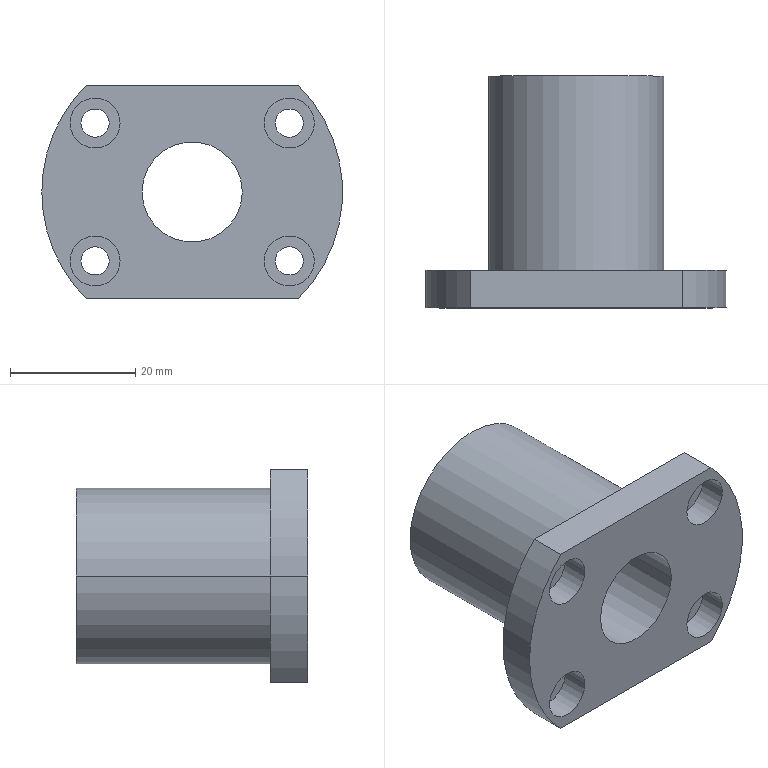Component | SolidWorks | FlangeLinearBearingLMH16UU-1 | 1 solid | 32 faces | box 48 x 37 x 34 mm | volume 19559 mm3 | cylinder 23 | plane 9 | commonest cylinder face diameters 8 x8 4.5 x8 48 x3 16 x2 28 x2
build123d program:
from build123d import *

# Parameters (mm, degrees)
BOSS_EXTRUDE1_DEPTH = 6
SKETCH3_R           = 14
BOSS_EXTRUDE2_DEPTH = 31
SKETCH4_R           = 8
CUT_EXTRUDE1_DEPTH  = 48.265
SKETCH5_R           = 2.25
CUT_EXTRUDE2_DEPTH  = 31
SKETCH6_R           = 4
CUT_EXTRUDE3_DEPTH  = 4.4


with BuildPart() as part:
    # Sketch1 → Boss-Extrude1 (new body)
    with BuildSketch(Plane(origin=(0, 0, 0), x_dir=(1, 0, 0), z_dir=(0, 1, 0))):
        with BuildLine():
            Line((-17, 16.941), (-17, -16.941))
            ThreePointArc((-17, -16.941), (0, -24), (17, -16.941))
            Line((17, -16.941), (17, 16.941))
            ThreePointArc((17, 16.941), (0, 24), (-17, 16.941))
        make_face()
    extrude(amount=BOSS_EXTRUDE1_DEPTH)

    # Sketch3 → Boss-Extrude2 (add)
    with BuildSketch(Plane(origin=(0, 6, 0), x_dir=(1, 0, 0), z_dir=(0, 1, 0))):
        with Locations(Location((0, 0, 0), (0, 0, 270))):
            Circle(SKETCH3_R)
    extrude(amount=BOSS_EXTRUDE2_DEPTH)

    # Sketch4 → Cut-Extrude1 (cut, through all)
    with BuildSketch(Plane(origin=(0, 37, 0), x_dir=(1, 0, 0), z_dir=(0, 1, 0))):
        with Locations(Location((0, 0, 0), (0, 0, 270))):
            Circle(SKETCH4_R)
    extrude(amount=-CUT_EXTRUDE1_DEPTH, mode=Mode.SUBTRACT)

    # Sketch5 → Cut-Extrude2 (cut)
    with BuildSketch(Plane.XZ):
        with Locations(Location((-11, 15.5, 0), (0, 0, 270))):
            Circle(SKETCH5_R)
        with Locations(Location((11, 15.5, 0), (0, 0, 270))):
            Circle(SKETCH5_R)
        with Locations(Location((11, -15.5, 0), (0, 0, 270))):
            Circle(SKETCH5_R)
        with Locations(Location((-11, -15.5, 0), (0, 0, 270))):
            Circle(SKETCH5_R)
    extrude(amount=-CUT_EXTRUDE2_DEPTH, mode=Mode.SUBTRACT)

    # Sketch6 → Cut-Extrude3 (cut)
    with BuildSketch(Plane.XZ):
        with Locations(Location((-11, 15.5, 0), (0, 0, 270))):
            Circle(SKETCH6_R)
        with Locations(Location((11, 15.5, 0), (0, 0, 270))):
            Circle(SKETCH6_R)
        with Locations(Location((11, -15.5, 0), (0, 0, 270))):
            Circle(SKETCH6_R)
        with Locations(Location((-11, -15.5, 0), (0, 0, 270))):
            Circle(SKETCH6_R)
    extrude(amount=-CUT_EXTRUDE3_DEPTH, mode=Mode.SUBTRACT)


solid = part.part

# Placed as in the assembly
solid = solid.moved(Location((32.2, 65.857, 29.75), (0, 90, 0)))
STEP:
#1=CARTESIAN_POINT('',(0.8149,2.766,1.604));
#2=VERTEX_POINT('',#1);
#3=CARTESIAN_POINT('',(0.5,2.766,1.604));
#4=VERTEX_POINT('',#3);
#5=CARTESIAN_POINT('',(0.6575,2.766,1.604));
#6=DIRECTION('',(0.,-1.,0.));
#7=DIRECTION('',(-1.,0.,0.));
#8=AXIS2_PLACEMENT_3D('',#5,#6,#7);
#9=CIRCLE('',#8,0.1575);
#10=EDGE_CURVE('',#2,#4,#9,.T.);
#11=ORIENTED_EDGE('',*,*,#10,.F.);
#12=CARTESIAN_POINT('',(0.8149,2.593,1.604));
#13=VERTEX_POINT('',#12);
#14=CARTESIAN_POINT('',(0.8149,2.766,1.604));
#15=DIRECTION('',(0.,-1.,0.));
#16=VECTOR('',#15,39.37);
#17=LINE('',#14,#16);
#18=EDGE_CURVE('',#2,#13,#17,.T.);
#19=ORIENTED_EDGE('',*,*,#18,.T.);
#20=CARTESIAN_POINT('',(0.5,2.593,1.604));
#21=VERTEX_POINT('',#20);
#22=CARTESIAN_POINT('',(0.6575,2.593,1.604));
#23=DIRECTION('',(0.,-1.,0.));
#24=DIRECTION('',(-1.,0.,0.));
#25=AXIS2_PLACEMENT_3D('',#22,#23,#24);
#26=CIRCLE('',#25,0.1575);
#27=EDGE_CURVE('',#13,#21,#26,.T.);
#28=ORIENTED_EDGE('',*,*,#27,.T.);
#29=CARTESIAN_POINT('',(0.5,2.766,1.604));
#30=DIRECTION('',(0.,-1.,0.));
#31=VECTOR('',#30,39.37);
#32=LINE('',#29,#31);
#33=EDGE_CURVE('',#4,#21,#32,.T.);
#34=ORIENTED_EDGE('',*,*,#33,.F.);
#35=EDGE_LOOP('',(#11,#19,#28,#34));
#36=FACE_OUTER_BOUND('',#35,.T.);
#37=CARTESIAN_POINT('',(0.6575,2.766,1.604));
#38=DIRECTION('',(0.,-1.,0.));
#39=DIRECTION('',(-1.,0.,0.));
#40=AXIS2_PLACEMENT_3D('',#37,#38,#39);
#41=CYLINDRICAL_SURFACE('',#40,0.1575);
#42=ADVANCED_FACE('',(#36),#41,.F.);
#43=CARTESIAN_POINT('',(0.8149,2.766,0.7382));
#44=VERTEX_POINT('',#43);
#45=CARTESIAN_POINT('',(0.5,2.766,0.7382));
#46=VERTEX_POINT('',#45);
#47=CARTESIAN_POINT('',(0.6575,2.766,0.7382));
#48=DIRECTION('',(0.,-1.,0.));
#49=DIRECTION('',(-1.,0.,0.));
#50=AXIS2_PLACEMENT_3D('',#47,#48,#49);
#51=CIRCLE('',#50,0.1575);
#52=EDGE_CURVE('',#44,#46,#51,.T.);
#53=ORIENTED_EDGE('',*,*,#52,.F.);
#54=CARTESIAN_POINT('',(0.8149,2.593,0.7382));
#55=VERTEX_POINT('',#54);
#56=CARTESIAN_POINT('',(0.8149,2.766,0.7382));
#57=DIRECTION('',(0.,-1.,0.));
#58=VECTOR('',#57,39.37);
#59=LINE('',#56,#58);
#60=EDGE_CURVE('',#44,#55,#59,.T.);
#61=ORIENTED_EDGE('',*,*,#60,.T.);
#62=CARTESIAN_POINT('',(0.5,2.593,0.7382));
#63=VERTEX_POINT('',#62);
#64=CARTESIAN_POINT('',(0.6575,2.593,0.7382));
#65=DIRECTION('',(0.,-1.,0.));
#66=DIRECTION('',(-1.,0.,0.));
#67=AXIS2_PLACEMENT_3D('',#64,#65,#66);
#68=CIRCLE('',#67,0.1575);
#69=EDGE_CURVE('',#55,#63,#68,.T.);
#70=ORIENTED_EDGE('',*,*,#69,.T.);
#71=CARTESIAN_POINT('',(0.5,2.766,0.7382));
#72=DIRECTION('',(0.,-1.,0.));
#73=VECTOR('',#72,39.37);
#74=LINE('',#71,#73);
#75=EDGE_CURVE('',#46,#63,#74,.T.);
#76=ORIENTED_EDGE('',*,*,#75,.F.);
#77=EDGE_LOOP('',(#53,#61,#70,#76));
#78=FACE_OUTER_BOUND('',#77,.T.);
#79=CARTESIAN_POINT('',(0.6575,2.766,0.7382));
#80=DIRECTION('',(0.,-1.,0.));
#81=DIRECTION('',(-1.,0.,0.));
#82=AXIS2_PLACEMENT_3D('',#79,#80,#81);
#83=CYLINDRICAL_SURFACE('',#82,0.1575);
#84=ADVANCED_FACE('',(#78),#83,.F.);
#85=CARTESIAN_POINT('',(2.035,2.766,0.7382));
#86=VERTEX_POINT('',#85);
#87=CARTESIAN_POINT('',(1.72,2.766,0.7382));
#88=VERTEX_POINT('',#87);
#89=CARTESIAN_POINT('',(1.878,2.766,0.7382));
#90=DIRECTION('',(0.,-1.,0.));
#91=DIRECTION('',(-1.,0.,0.));
#92=AXIS2_PLACEMENT_3D('',#89,#90,#91);
#93=CIRCLE('',#92,0.1575);
#94=EDGE_CURVE('',#86,#88,#93,.T.);
#95=ORIENTED_EDGE('',*,*,#94,.F.);
#96=CARTESIAN_POINT('',(2.035,2.593,0.7382));
#97=VERTEX_POINT('',#96);
#98=CARTESIAN_POINT('',(2.035,2.766,0.7382));
#99=DIRECTION('',(0.,-1.,0.));
#100=VECTOR('',#99,39.37);
#101=LINE('',#98,#100);
#102=EDGE_CURVE('',#86,#97,#101,.T.);
#103=ORIENTED_EDGE('',*,*,#102,.T.);
#104=CARTESIAN_POINT('',(1.72,2.593,0.7382));
#105=VERTEX_POINT('',#104);
#106=CARTESIAN_POINT('',(1.878,2.593,0.7382));
#107=DIRECTION('',(0.,-1.,0.));
#108=DIRECTION('',(-1.,0.,0.));
#109=AXIS2_PLACEMENT_3D('',#106,#107,#108);
#110=CIRCLE('',#109,0.1575);
#111=EDGE_CURVE('',#97,#105,#110,.T.);
#112=ORIENTED_EDGE('',*,*,#111,.T.);
#113=CARTESIAN_POINT('',(1.72,2.766,0.7382));
#114=DIRECTION('',(0.,-1.,0.));
#115=VECTOR('',#114,39.37);
#116=LINE('',#113,#115);
#117=EDGE_CURVE('',#88,#105,#116,.T.);
#118=ORIENTED_EDGE('',*,*,#117,.F.);
#119=EDGE_LOOP('',(#95,#103,#112,#118));
#120=FACE_OUTER_BOUND('',#119,.T.);
#121=CARTESIAN_POINT('',(1.878,2.766,0.7382));
#122=DIRECTION('',(0.,-1.,0.));
#123=DIRECTION('',(-1.,0.,0.));
#124=AXIS2_PLACEMENT_3D('',#121,#122,#123);
#125=CYLINDRICAL_SURFACE('',#124,0.1575);
#126=ADVANCED_FACE('',(#120),#125,.F.);
#127=CARTESIAN_POINT('',(2.035,2.766,1.604));
#128=VERTEX_POINT('',#127);
#129=CARTESIAN_POINT('',(1.72,2.766,1.604));
#130=VERTEX_POINT('',#129);
#131=CARTESIAN_POINT('',(1.878,2.766,1.604));
#132=DIRECTION('',(0.,-1.,0.));
#133=DIRECTION('',(-1.,0.,0.));
#134=AXIS2_PLACEMENT_3D('',#131,#132,#133);
#135=CIRCLE('',#134,0.1575);
#136=EDGE_CURVE('',#128,#130,#135,.T.);
#137=ORIENTED_EDGE('',*,*,#136,.F.);
#138=CARTESIAN_POINT('',(2.035,2.593,1.604));
#139=VERTEX_POINT('',#138);
#140=CARTESIAN_POINT('',(2.035,2.766,1.604));
#141=DIRECTION('',(0.,-1.,0.));
#142=VECTOR('',#141,39.37);
#143=LINE('',#140,#142);
#144=EDGE_CURVE('',#128,#139,#143,.T.);
#145=ORIENTED_EDGE('',*,*,#144,.T.);
#146=CARTESIAN_POINT('',(1.72,2.593,1.604));
#147=VERTEX_POINT('',#146);
#148=CARTESIAN_POINT('',(1.878,2.593,1.604));
#149=DIRECTION('',(0.,-1.,0.));
#150=DIRECTION('',(-1.,0.,0.));
#151=AXIS2_PLACEMENT_3D('',#148,#149,#150);
#152=CIRCLE('',#151,0.1575);
#153=EDGE_CURVE('',#139,#147,#152,.T.);
#154=ORIENTED_EDGE('',*,*,#153,.T.);
#155=CARTESIAN_POINT('',(1.72,2.766,1.604));
#156=DIRECTION('',(0.,-1.,0.));
#157=VECTOR('',#156,39.37);
#158=LINE('',#155,#157);
#159=EDGE_CURVE('',#130,#147,#158,.T.);
#160=ORIENTED_EDGE('',*,*,#159,.F.);
#161=EDGE_LOOP('',(#137,#145,#154,#160));
#162=FACE_OUTER_BOUND('',#161,.T.);
#163=CARTESIAN_POINT('',(1.878,2.766,1.604));
#164=DIRECTION('',(0.,-1.,0.));
#165=DIRECTION('',(-1.,0.,0.));
#166=AXIS2_PLACEMENT_3D('',#163,#164,#165);
#167=CYLINDRICAL_SURFACE('',#166,0.1575);
#168=ADVANCED_FACE('',(#162),#167,.F.);
#169=CARTESIAN_POINT('',(0.9527,2.593,1.171));
#170=VERTEX_POINT('',#169);
#171=CARTESIAN_POINT('',(1.583,2.593,1.171));
#172=VERTEX_POINT('',#171);
#173=CARTESIAN_POINT('',(1.268,2.593,1.171));
#174=DIRECTION('',(0.,1.,0.));
#175=DIRECTION('',(1.,0.,0.));
#176=AXIS2_PLACEMENT_3D('',#173,#174,#175);
#177=CIRCLE('',#176,0.315);
#178=EDGE_CURVE('',#170,#172,#177,.T.);
#179=ORIENTED_EDGE('',*,*,#178,.F.);
#180=CARTESIAN_POINT('',(0.9527,4.049,1.171));
#181=VERTEX_POINT('',#180);
#182=CARTESIAN_POINT('',(0.9527,2.593,1.171));
#183=DIRECTION('',(0.,1.,0.));
#184=VECTOR('',#183,39.37);
#185=LINE('',#182,#184);
#186=EDGE_CURVE('',#170,#181,#185,.T.);
#187=ORIENTED_EDGE('',*,*,#186,.T.);
#188=CARTESIAN_POINT('',(1.583,4.049,1.171));
#189=VERTEX_POINT('',#188);
#190=CARTESIAN_POINT('',(1.268,4.049,1.171));
#191=DIRECTION('',(0.,1.,0.));
#192=DIRECTION('',(1.,0.,0.));
#193=AXIS2_PLACEMENT_3D('',#190,#191,#192);
#194=CIRCLE('',#193,0.315);
#195=EDGE_CURVE('',#181,#189,#194,.T.);
#196=ORIENTED_EDGE('',*,*,#195,.T.);
#197=CARTESIAN_POINT('',(1.583,2.593,1.171));
#198=DIRECTION('',(0.,1.,0.));
#199=VECTOR('',#198,39.37);
#200=LINE('',#197,#199);
#201=EDGE_CURVE('',#172,#189,#200,.T.);
#202=ORIENTED_EDGE('',*,*,#201,.F.);
#203=EDGE_LOOP('',(#179,#187,#196,#202));
#204=FACE_OUTER_BOUND('',#203,.T.);
#205=CARTESIAN_POINT('',(1.268,2.593,1.171));
#206=DIRECTION('',(0.,1.,0.));
#207=DIRECTION('',(1.,0.,0.));
#208=AXIS2_PLACEMENT_3D('',#205,#206,#207);
#209=CYLINDRICAL_SURFACE('',#208,0.315);
#210=ADVANCED_FACE('',(#204),#209,.F.);
#211=CARTESIAN_POINT('',(1.819,4.049,1.171));
#212=VERTEX_POINT('',#211);
#213=CARTESIAN_POINT('',(0.7165,4.049,1.171));
#214=VERTEX_POINT('',#213);
#215=CARTESIAN_POINT('',(1.268,4.049,1.171));
#216=DIRECTION('',(0.,1.,0.));
#217=DIRECTION('',(1.,0.,0.));
#218=AXIS2_PLACEMENT_3D('',#215,#216,#217);
#219=CIRCLE('',#218,0.5512);
#220=EDGE_CURVE('',#212,#214,#219,.T.);
#221=ORIENTED_EDGE('',*,*,#220,.F.);
#222=CARTESIAN_POINT('',(1.819,2.829,1.171));
#223=VERTEX_POINT('',#222);
#224=CARTESIAN_POINT('',(1.819,4.049,1.171));
#225=DIRECTION('',(0.,-1.,0.));
#226=VECTOR('',#225,39.37);
#227=LINE('',#224,#226);
#228=EDGE_CURVE('',#212,#223,#227,.T.);
#229=ORIENTED_EDGE('',*,*,#228,.T.);
#230=CARTESIAN_POINT('',(0.7165,2.829,1.171));
#231=VERTEX_POINT('',#230);
#232=CARTESIAN_POINT('',(1.268,2.829,1.171));
#233=DIRECTION('',(0.,1.,0.));
#234=DIRECTION('',(1.,0.,0.));
#235=AXIS2_PLACEMENT_3D('',#232,#233,#234);
#236=CIRCLE('',#235,0.5512);
#237=EDGE_CURVE('',#223,#231,#236,.T.);
#238=ORIENTED_EDGE('',*,*,#237,.T.);
#239=CARTESIAN_POINT('',(0.7165,4.049,1.171));
#240=DIRECTION('',(0.,-1.,0.));
#241=VECTOR('',#240,39.37);
#242=LINE('',#239,#241);
#243=EDGE_CURVE('',#214,#231,#242,.T.);
#244=ORIENTED_EDGE('',*,*,#243,.F.);
#245=EDGE_LOOP('',(#221,#229,#238,#244));
#246=FACE_OUTER_BOUND('',#245,.T.);
#247=CARTESIAN_POINT('',(1.268,4.049,1.171));
#248=DIRECTION('',(0.,-1.,0.));
#249=DIRECTION('',(-1.,0.,-0.));
#250=AXIS2_PLACEMENT_3D('',#247,#248,#249);
#251=CYLINDRICAL_SURFACE('',#250,0.5512);
#252=ADVANCED_FACE('',(#246),#251,.T.);
#253=CARTESIAN_POINT('',(0.3228,2.829,1.171));
#254=VERTEX_POINT('',#253);
#255=CARTESIAN_POINT('',(0.6007,2.829,1.841));
#256=VERTEX_POINT('',#255);
#257=CARTESIAN_POINT('',(1.268,2.829,1.171));
#258=DIRECTION('',(0.,1.,0.));
#259=DIRECTION('',(1.,0.,0.));
#260=AXIS2_PLACEMENT_3D('',#257,#258,#259);
#261=CIRCLE('',#260,0.9449);
#262=EDGE_CURVE('',#254,#256,#261,.T.);
#263=ORIENTED_EDGE('',*,*,#262,.F.);
#264=CARTESIAN_POINT('',(0.3228,2.593,1.171));
#265=VERTEX_POINT('',#264);
#266=CARTESIAN_POINT('',(0.3228,2.829,1.171));
#267=DIRECTION('',(0.,-1.,0.));
#268=VECTOR('',#267,39.37);
#269=LINE('',#266,#268);
#270=EDGE_CURVE('',#254,#265,#269,.T.);
#271=ORIENTED_EDGE('',*,*,#270,.T.);
#272=CARTESIAN_POINT('',(0.6007,2.593,1.841));
#273=VERTEX_POINT('',#272);
#274=CARTESIAN_POINT('',(1.268,2.593,1.171));
#275=DIRECTION('',(0.,1.,0.));
#276=DIRECTION('',(1.,0.,0.));
#277=AXIS2_PLACEMENT_3D('',#274,#275,#276);
#278=CIRCLE('',#277,0.9449);
#279=EDGE_CURVE('',#265,#273,#278,.T.);
#280=ORIENTED_EDGE('',*,*,#279,.T.);
#281=CARTESIAN_POINT('',(0.6007,2.829,1.841));
#282=DIRECTION('',(0.,-1.,0.));
#283=VECTOR('',#282,39.37);
#284=LINE('',#281,#283);
#285=EDGE_CURVE('',#256,#273,#284,.T.);
#286=ORIENTED_EDGE('',*,*,#285,.F.);
#287=EDGE_LOOP('',(#263,#271,#280,#286));
#288=FACE_OUTER_BOUND('',#287,.T.);
#289=CARTESIAN_POINT('',(1.268,2.829,1.171));
#290=DIRECTION('',(0.,-1.,0.));
#291=DIRECTION('',(-1.,0.,-0.));
#292=AXIS2_PLACEMENT_3D('',#289,#290,#291);
#293=CYLINDRICAL_SURFACE('',#292,0.9449);
#294=ADVANCED_FACE('',(#288),#293,.T.);
#295=CARTESIAN_POINT('',(1.789,2.829,1.604));
#296=VERTEX_POINT('',#295);
#297=CARTESIAN_POINT('',(1.967,2.829,1.604));
#298=VERTEX_POINT('',#297);
#299=CARTESIAN_POINT('',(1.878,2.829,1.604));
#300=DIRECTION('',(0.,1.,0.));
#301=DIRECTION('',(1.,0.,0.));
#302=AXIS2_PLACEMENT_3D('',#299,#300,#301);
#303=CIRCLE('',#302,0.08858);
#304=EDGE_CURVE('',#296,#298,#303,.T.);
#305=ORIENTED_EDGE('',*,*,#304,.T.);
#306=CARTESIAN_POINT('',(1.967,2.766,1.604));
#307=VERTEX_POINT('',#306);
#308=CARTESIAN_POINT('',(1.967,3.813,1.604));
#309=DIRECTION('',(0.,-1.,0.));
#310=VECTOR('',#309,39.37);
#311=LINE('',#308,#310);
#312=EDGE_CURVE('',#298,#307,#311,.T.);
#313=ORIENTED_EDGE('',*,*,#312,.T.);
#314=CARTESIAN_POINT('',(1.789,2.766,1.604));
#315=VERTEX_POINT('',#314);
#316=CARTESIAN_POINT('',(1.878,2.766,1.604));
#317=DIRECTION('',(0.,1.,0.));
#318=DIRECTION('',(-1.,0.,0.));
#319=AXIS2_PLACEMENT_3D('',#316,#317,#318);
#320=CIRCLE('',#319,0.08858);
#321=EDGE_CURVE('',#315,#307,#320,.T.);
#322=ORIENTED_EDGE('',*,*,#321,.F.);
#323=CARTESIAN_POINT('',(1.789,3.813,1.604));
#324=DIRECTION('',(0.,-1.,0.));
#325=VECTOR('',#324,39.37);
#326=LINE('',#323,#325);
#327=EDGE_CURVE('',#296,#315,#326,.T.);
#328=ORIENTED_EDGE('',*,*,#327,.F.);
#329=EDGE_LOOP('',(#305,#313,#322,#328));
#330=FACE_OUTER_BOUND('',#329,.T.);
#331=CARTESIAN_POINT('',(1.878,3.813,1.604));
#332=DIRECTION('',(0.,-1.,0.));
#333=DIRECTION('',(-1.,0.,0.));
#334=AXIS2_PLACEMENT_3D('',#331,#332,#333);
#335=CYLINDRICAL_SURFACE('',#334,0.08858);
#336=ADVANCED_FACE('',(#330),#335,.F.);
#337=CARTESIAN_POINT('',(1.789,2.829,0.7382));
#338=VERTEX_POINT('',#337);
#339=CARTESIAN_POINT('',(1.967,2.829,0.7382));
#340=VERTEX_POINT('',#339);
#341=CARTESIAN_POINT('',(1.878,2.829,0.7382));
#342=DIRECTION('',(0.,1.,0.));
#343=DIRECTION('',(1.,0.,0.));
#344=AXIS2_PLACEMENT_3D('',#341,#342,#343);
#345=CIRCLE('',#344,0.08858);
#346=EDGE_CURVE('',#338,#340,#345,.T.);
#347=ORIENTED_EDGE('',*,*,#346,.T.);
#348=CARTESIAN_POINT('',(1.967,2.766,0.7382));
#349=VERTEX_POINT('',#348);
#350=CARTESIAN_POINT('',(1.967,3.813,0.7382));
#351=DIRECTION('',(0.,-1.,0.));
#352=VECTOR('',#351,39.37);
#353=LINE('',#350,#352);
#354=EDGE_CURVE('',#340,#349,#353,.T.);
#355=ORIENTED_EDGE('',*,*,#354,.T.);
#356=CARTESIAN_POINT('',(1.789,2.766,0.7382));
#357=VERTEX_POINT('',#356);
#358=CARTESIAN_POINT('',(1.878,2.766,0.7382));
#359=DIRECTION('',(0.,1.,0.));
#360=DIRECTION('',(-1.,0.,0.));
#361=AXIS2_PLACEMENT_3D('',#358,#359,#360);
#362=CIRCLE('',#361,0.08858);
#363=EDGE_CURVE('',#357,#349,#362,.T.);
#364=ORIENTED_EDGE('',*,*,#363,.F.);
#365=CARTESIAN_POINT('',(1.789,3.813,0.7382));
#366=DIRECTION('',(0.,-1.,0.));
#367=VECTOR('',#366,39.37);
#368=LINE('',#365,#367);
#369=EDGE_CURVE('',#338,#357,#368,.T.);
#370=ORIENTED_EDGE('',*,*,#369,.F.);
#371=EDGE_LOOP('',(#347,#355,#364,#370));
#372=FACE_OUTER_BOUND('',#371,.T.);
#373=CARTESIAN_POINT('',(1.878,3.813,0.7382));
#374=DIRECTION('',(0.,-1.,0.));
#375=DIRECTION('',(-1.,0.,0.));
#376=AXIS2_PLACEMENT_3D('',#373,#374,#375);
#377=CYLINDRICAL_SURFACE('',#376,0.08858);
#378=ADVANCED_FACE('',(#372),#377,.F.);
#379=CARTESIAN_POINT('',(0.5689,2.829,0.7382));
#380=VERTEX_POINT('',#379);
#381=CARTESIAN_POINT('',(0.746,2.829,0.7382));
#382=VERTEX_POINT('',#381);
#383=CARTESIAN_POINT('',(0.6575,2.829,0.7382));
#384=DIRECTION('',(0.,1.,0.));
#385=DIRECTION('',(1.,0.,0.));
#386=AXIS2_PLACEMENT_3D('',#383,#384,#385);
#387=CIRCLE('',#386,0.08858);
#388=EDGE_CURVE('',#380,#382,#387,.T.);
#389=ORIENTED_EDGE('',*,*,#388,.T.);
#390=CARTESIAN_POINT('',(0.746,2.766,0.7382));
#391=VERTEX_POINT('',#390);
#392=CARTESIAN_POINT('',(0.746,3.813,0.7382));
#393=DIRECTION('',(0.,-1.,0.));
#394=VECTOR('',#393,39.37);
#395=LINE('',#392,#394);
#396=EDGE_CURVE('',#382,#391,#395,.T.);
#397=ORIENTED_EDGE('',*,*,#396,.T.);
#398=CARTESIAN_POINT('',(0.5689,2.766,0.7382));
#399=VERTEX_POINT('',#398);
#400=CARTESIAN_POINT('',(0.6575,2.766,0.7382));
#401=DIRECTION('',(0.,1.,0.));
#402=DIRECTION('',(-1.,0.,0.));
#403=AXIS2_PLACEMENT_3D('',#400,#401,#402);
#404=CIRCLE('',#403,0.08858);
#405=EDGE_CURVE('',#399,#391,#404,.T.);
#406=ORIENTED_EDGE('',*,*,#405,.F.);
#407=CARTESIAN_POINT('',(0.5689,3.813,0.7382));
#408=DIRECTION('',(0.,-1.,0.));
#409=VECTOR('',#408,39.37);
#410=LINE('',#407,#409);
#411=EDGE_CURVE('',#380,#399,#410,.T.);
#412=ORIENTED_EDGE('',*,*,#411,.F.);
#413=EDGE_LOOP('',(#389,#397,#406,#412));
#414=FACE_OUTER_BOUND('',#413,.T.);
#415=CARTESIAN_POINT('',(0.6575,3.813,0.7382));
#416=DIRECTION('',(0.,-1.,0.));
#417=DIRECTION('',(-1.,0.,0.));
#418=AXIS2_PLACEMENT_3D('',#415,#416,#417);
#419=CYLINDRICAL_SURFACE('',#418,0.08858);
#420=ADVANCED_FACE('',(#414),#419,.F.);
#421=CARTESIAN_POINT('',(0.5689,2.829,1.604));
#422=VERTEX_POINT('',#421);
#423=CARTESIAN_POINT('',(0.746,2.829,1.604));
#424=VERTEX_POINT('',#423);
#425=CARTESIAN_POINT('',(0.6575,2.829,1.604));
#426=DIRECTION('',(0.,1.,0.));
#427=DIRECTION('',(1.,0.,0.));
#428=AXIS2_PLACEMENT_3D('',#425,#426,#427);
#429=CIRCLE('',#428,0.08858);
#430=EDGE_CURVE('',#422,#424,#429,.T.);
#431=ORIENTED_EDGE('',*,*,#430,.T.);
#432=CARTESIAN_POINT('',(0.746,2.766,1.604));
#433=VERTEX_POINT('',#432);
#434=CARTESIAN_POINT('',(0.746,3.813,1.604));
#435=DIRECTION('',(0.,-1.,0.));
#436=VECTOR('',#435,39.37);
#437=LINE('',#434,#436);
#438=EDGE_CURVE('',#424,#433,#437,.T.);
#439=ORIENTED_EDGE('',*,*,#438,.T.);
#440=CARTESIAN_POINT('',(0.5689,2.766,1.604));
#441=VERTEX_POINT('',#440);
#442=CARTESIAN_POINT('',(0.6575,2.766,1.604));
#443=DIRECTION('',(0.,1.,0.));
#444=DIRECTION('',(-1.,0.,0.));
#445=AXIS2_PLACEMENT_3D('',#442,#443,#444);
#446=CIRCLE('',#445,0.08858);
#447=EDGE_CURVE('',#441,#433,#446,.T.);
#448=ORIENTED_EDGE('',*,*,#447,.F.);
#449=CARTESIAN_POINT('',(0.5689,3.813,1.604));
#450=DIRECTION('',(0.,-1.,0.));
#451=VECTOR('',#450,39.37);
#452=LINE('',#449,#451);
#453=EDGE_CURVE('',#422,#441,#452,.T.);
#454=ORIENTED_EDGE('',*,*,#453,.F.);
#455=EDGE_LOOP('',(#431,#439,#448,#454));
#456=FACE_OUTER_BOUND('',#455,.T.);
#457=CARTESIAN_POINT('',(0.6575,3.813,1.604));
#458=DIRECTION('',(0.,-1.,0.));
#459=DIRECTION('',(-1.,0.,0.));
#460=AXIS2_PLACEMENT_3D('',#457,#458,#459);
#461=CYLINDRICAL_SURFACE('',#460,0.08858);
#462=ADVANCED_FACE('',(#456),#461,.F.);
#463=ORIENTED_EDGE('',*,*,#438,.F.);
#464=CARTESIAN_POINT('',(0.6575,2.829,1.604));
#465=DIRECTION('',(0.,1.,0.));
#466=DIRECTION('',(1.,0.,0.));
#467=AXIS2_PLACEMENT_3D('',#464,#465,#466);
#468=CIRCLE('',#467,0.08858);
#469=EDGE_CURVE('',#424,#422,#468,.T.);
#470=ORIENTED_EDGE('',*,*,#469,.T.);
#471=ORIENTED_EDGE('',*,*,#453,.T.);
#472=CARTESIAN_POINT('',(0.6575,2.766,1.604));
#473=DIRECTION('',(0.,1.,0.));
#474=DIRECTION('',(-1.,0.,0.));
#475=AXIS2_PLACEMENT_3D('',#472,#473,#474);
#476=CIRCLE('',#475,0.08858);
#477=EDGE_CURVE('',#433,#441,#476,.T.);
#478=ORIENTED_EDGE('',*,*,#477,.F.);
#479=EDGE_LOOP('',(#463,#470,#471,#478));
#480=FACE_OUTER_BOUND('',#479,.T.);
#481=CARTESIAN_POINT('',(0.6575,3.813,1.604));
#482=DIRECTION('',(0.,-1.,0.));
#483=DIRECTION('',(-1.,0.,0.));
#484=AXIS2_PLACEMENT_3D('',#481,#482,#483);
#485=CYLINDRICAL_SURFACE('',#484,0.08858);
#486=ADVANCED_FACE('',(#480),#485,.F.);
#487=ORIENTED_EDGE('',*,*,#396,.F.);
#488=CARTESIAN_POINT('',(0.6575,2.829,0.7382));
#489=DIRECTION('',(0.,1.,0.));
#490=DIRECTION('',(1.,0.,0.));
#491=AXIS2_PLACEMENT_3D('',#488,#489,#490);
#492=CIRCLE('',#491,0.08858);
#493=EDGE_CURVE('',#382,#380,#492,.T.);
#494=ORIENTED_EDGE('',*,*,#493,.T.);
#495=ORIENTED_EDGE('',*,*,#411,.T.);
#496=CARTESIAN_POINT('',(0.6575,2.766,0.7382));
#497=DIRECTION('',(0.,1.,0.));
#498=DIRECTION('',(-1.,0.,0.));
#499=AXIS2_PLACEMENT_3D('',#496,#497,#498);
#500=CIRCLE('',#499,0.08858);
#501=EDGE_CURVE('',#391,#399,#500,.T.);
#502=ORIENTED_EDGE('',*,*,#501,.F.);
#503=EDGE_LOOP('',(#487,#494,#495,#502));
#504=FACE_OUTER_BOUND('',#503,.T.);
#505=CARTESIAN_POINT('',(0.6575,3.813,0.7382));
#506=DIRECTION('',(0.,-1.,0.));
#507=DIRECTION('',(-1.,0.,0.));
#508=AXIS2_PLACEMENT_3D('',#505,#506,#507);
#509=CYLINDRICAL_SURFACE('',#508,0.08858);
#510=ADVANCED_FACE('',(#504),#509,.F.);
#511=ORIENTED_EDGE('',*,*,#354,.F.);
#512=CARTESIAN_POINT('',(1.878,2.829,0.7382));
#513=DIRECTION('',(0.,1.,0.));
#514=DIRECTION('',(1.,0.,0.));
#515=AXIS2_PLACEMENT_3D('',#512,#513,#514);
#516=CIRCLE('',#515,0.08858);
#517=EDGE_CURVE('',#340,#338,#516,.T.);
#518=ORIENTED_EDGE('',*,*,#517,.T.);
#519=ORIENTED_EDGE('',*,*,#369,.T.);
#520=CARTESIAN_POINT('',(1.878,2.766,0.7382));
#521=DIRECTION('',(0.,1.,0.));
#522=DIRECTION('',(-1.,0.,0.));
#523=AXIS2_PLACEMENT_3D('',#520,#521,#522);
#524=CIRCLE('',#523,0.08858);
#525=EDGE_CURVE('',#349,#357,#524,.T.);
#526=ORIENTED_EDGE('',*,*,#525,.F.);
#527=EDGE_LOOP('',(#511,#518,#519,#526));
#528=FACE_OUTER_BOUND('',#527,.T.);
#529=CARTESIAN_POINT('',(1.878,3.813,0.7382));
#530=DIRECTION('',(0.,-1.,0.));
#531=DIRECTION('',(-1.,0.,0.));
#532=AXIS2_PLACEMENT_3D('',#529,#530,#531);
#533=CYLINDRICAL_SURFACE('',#532,0.08858);
#534=ADVANCED_FACE('',(#528),#533,.F.);
#535=ORIENTED_EDGE('',*,*,#312,.F.);
#536=CARTESIAN_POINT('',(1.878,2.829,1.604));
#537=DIRECTION('',(0.,1.,0.));
#538=DIRECTION('',(1.,0.,0.));
#539=AXIS2_PLACEMENT_3D('',#536,#537,#538);
#540=CIRCLE('',#539,0.08858);
#541=EDGE_CURVE('',#298,#296,#540,.T.);
#542=ORIENTED_EDGE('',*,*,#541,.T.);
#543=ORIENTED_EDGE('',*,*,#327,.T.);
#544=CARTESIAN_POINT('',(1.878,2.766,1.604));
#545=DIRECTION('',(0.,1.,0.));
#546=DIRECTION('',(-1.,0.,0.));
#547=AXIS2_PLACEMENT_3D('',#544,#545,#546);
#548=CIRCLE('',#547,0.08858);
#549=EDGE_CURVE('',#307,#315,#548,.T.);
#550=ORIENTED_EDGE('',*,*,#549,.F.);
#551=EDGE_LOOP('',(#535,#542,#543,#550));
#552=FACE_OUTER_BOUND('',#551,.T.);
#553=CARTESIAN_POINT('',(1.878,3.813,1.604));
#554=DIRECTION('',(0.,-1.,0.));
#555=DIRECTION('',(-1.,0.,0.));
#556=AXIS2_PLACEMENT_3D('',#553,#554,#555);
#557=CYLINDRICAL_SURFACE('',#556,0.08858);
#558=ADVANCED_FACE('',(#552),#557,.F.);
#559=ORIENTED_EDGE('',*,*,#270,.F.);
#560=CARTESIAN_POINT('',(0.6007,2.829,0.502));
#561=VERTEX_POINT('',#560);
#562=CARTESIAN_POINT('',(1.268,2.829,1.171));
#563=DIRECTION('',(0.,1.,0.));
#564=DIRECTION('',(1.,0.,0.));
#565=AXIS2_PLACEMENT_3D('',#562,#563,#564);
#566=CIRCLE('',#565,0.9449);
#567=EDGE_CURVE('',#561,#254,#566,.T.);
#568=ORIENTED_EDGE('',*,*,#567,.F.);
#569=CARTESIAN_POINT('',(0.6007,2.593,0.502));
#570=VERTEX_POINT('',#569);
#571=CARTESIAN_POINT('',(0.6007,2.829,0.502));
#572=DIRECTION('',(0.,-1.,0.));
#573=VECTOR('',#572,39.37);
#574=LINE('',#571,#573);
#575=EDGE_CURVE('',#561,#570,#574,.T.);
#576=ORIENTED_EDGE('',*,*,#575,.T.);
#577=CARTESIAN_POINT('',(1.268,2.593,1.171));
#578=DIRECTION('',(0.,1.,0.));
#579=DIRECTION('',(1.,0.,0.));
#580=AXIS2_PLACEMENT_3D('',#577,#578,#579);
#581=CIRCLE('',#580,0.9449);
#582=EDGE_CURVE('',#570,#265,#581,.T.);
#583=ORIENTED_EDGE('',*,*,#582,.T.);
#584=EDGE_LOOP('',(#559,#568,#576,#583));
#585=FACE_OUTER_BOUND('',#584,.T.);
#586=CARTESIAN_POINT('',(1.268,2.829,1.171));
#587=DIRECTION('',(0.,-1.,0.));
#588=DIRECTION('',(-1.,0.,-0.));
#589=AXIS2_PLACEMENT_3D('',#586,#587,#588);
#590=CYLINDRICAL_SURFACE('',#589,0.9449);
#591=ADVANCED_FACE('',(#585),#590,.T.);
#592=CARTESIAN_POINT('',(1.935,2.593,1.841));
#593=VERTEX_POINT('',#592);
#594=CARTESIAN_POINT('',(0.6007,2.593,1.841));
#595=DIRECTION('',(1.,0.,-0.));
#596=VECTOR('',#595,39.37);
#597=LINE('',#594,#596);
#598=EDGE_CURVE('',#273,#593,#597,.T.);
#599=ORIENTED_EDGE('',*,*,#598,.T.);
#600=CARTESIAN_POINT('',(1.935,2.829,1.841));
#601=VERTEX_POINT('',#600);
#602=CARTESIAN_POINT('',(1.935,2.829,1.841));
#603=DIRECTION('',(0.,-1.,0.));
#604=VECTOR('',#603,39.37);
#605=LINE('',#602,#604);
#606=EDGE_CURVE('',#601,#593,#605,.T.);
#607=ORIENTED_EDGE('',*,*,#606,.F.);
#608=CARTESIAN_POINT('',(0.6007,2.829,1.841));
#609=DIRECTION('',(1.,0.,-0.));
#610=VECTOR('',#609,39.37);
#611=LINE('',#608,#610);
#612=EDGE_CURVE('',#256,#601,#611,.T.);
#613=ORIENTED_EDGE('',*,*,#612,.F.);
#614=ORIENTED_EDGE('',*,*,#285,.T.);
#615=EDGE_LOOP('',(#599,#607,#613,#614));
#616=FACE_OUTER_BOUND('',#615,.T.);
#617=CARTESIAN_POINT('',(0.6007,2.829,1.841));
#618=DIRECTION('',(-0.,0.,-1.));
#619=DIRECTION('',(-1.,0.,0.));
#620=AXIS2_PLACEMENT_3D('',#617,#618,#619);
#621=PLANE('',#620);
#622=ADVANCED_FACE('',(#616),#621,.F.);
#623=CARTESIAN_POINT('',(1.935,2.593,0.502));
#624=VERTEX_POINT('',#623);
#625=CARTESIAN_POINT('',(1.268,2.593,1.171));
#626=DIRECTION('',(0.,1.,0.));
#627=DIRECTION('',(1.,0.,0.));
#628=AXIS2_PLACEMENT_3D('',#625,#626,#627);
#629=CIRCLE('',#628,0.9449);
#630=EDGE_CURVE('',#593,#624,#629,.T.);
#631=ORIENTED_EDGE('',*,*,#630,.T.);
#632=CARTESIAN_POINT('',(1.935,2.829,0.502));
#633=VERTEX_POINT('',#632);
#634=CARTESIAN_POINT('',(1.935,2.829,0.502));
#635=DIRECTION('',(0.,-1.,0.));
#636=VECTOR('',#635,39.37);
#637=LINE('',#634,#636);
#638=EDGE_CURVE('',#633,#624,#637,.T.);
#639=ORIENTED_EDGE('',*,*,#638,.F.);
#640=CARTESIAN_POINT('',(1.268,2.829,1.171));
#641=DIRECTION('',(0.,1.,0.));
#642=DIRECTION('',(1.,0.,0.));
#643=AXIS2_PLACEMENT_3D('',#640,#641,#642);
#644=CIRCLE('',#643,0.9449);
#645=EDGE_CURVE('',#601,#633,#644,.T.);
#646=ORIENTED_EDGE('',*,*,#645,.F.);
#647=ORIENTED_EDGE('',*,*,#606,.T.);
#648=EDGE_LOOP('',(#631,#639,#646,#647));
#649=FACE_OUTER_BOUND('',#648,.T.);
#650=CARTESIAN_POINT('',(1.268,2.829,1.171));
#651=DIRECTION('',(0.,-1.,0.));
#652=DIRECTION('',(-1.,0.,-0.));
#653=AXIS2_PLACEMENT_3D('',#650,#651,#652);
#654=CYLINDRICAL_SURFACE('',#653,0.9449);
#655=ADVANCED_FACE('',(#649),#654,.T.);
#656=CARTESIAN_POINT('',(0.6007,2.593,0.502));
#657=DIRECTION('',(-1.,0.,-0.));
#658=VECTOR('',#657,39.37);
#659=LINE('',#656,#658);
#660=EDGE_CURVE('',#624,#570,#659,.T.);
#661=ORIENTED_EDGE('',*,*,#660,.T.);
#662=ORIENTED_EDGE('',*,*,#575,.F.);
#663=CARTESIAN_POINT('',(0.6007,2.829,0.502));
#664=DIRECTION('',(-1.,0.,-0.));
#665=VECTOR('',#664,39.37);
#666=LINE('',#663,#665);
#667=EDGE_CURVE('',#633,#561,#666,.T.);
#668=ORIENTED_EDGE('',*,*,#667,.F.);
#669=ORIENTED_EDGE('',*,*,#638,.T.);
#670=EDGE_LOOP('',(#661,#662,#668,#669));
#671=FACE_OUTER_BOUND('',#670,.T.);
#672=CARTESIAN_POINT('',(0.6007,2.829,0.502));
#673=DIRECTION('',(-0.,0.,1.));
#674=DIRECTION('',(1.,0.,0.));
#675=AXIS2_PLACEMENT_3D('',#672,#673,#674);
#676=PLANE('',#675);
#677=ADVANCED_FACE('',(#671),#676,.F.);
#678=ORIENTED_EDGE('',*,*,#346,.F.);
#679=ORIENTED_EDGE('',*,*,#517,.F.);
#680=EDGE_LOOP('',(#678,#679));
#681=FACE_BOUND('',#680,.T.);
#682=ORIENTED_EDGE('',*,*,#388,.F.);
#683=ORIENTED_EDGE('',*,*,#493,.F.);
#684=EDGE_LOOP('',(#682,#683));
#685=FACE_BOUND('',#684,.T.);
#686=ORIENTED_EDGE('',*,*,#430,.F.);
#687=ORIENTED_EDGE('',*,*,#469,.F.);
#688=EDGE_LOOP('',(#686,#687));
#689=FACE_BOUND('',#688,.T.);
#690=ORIENTED_EDGE('',*,*,#304,.F.);
#691=ORIENTED_EDGE('',*,*,#541,.F.);
#692=EDGE_LOOP('',(#690,#691));
#693=FACE_BOUND('',#692,.T.);
#694=CARTESIAN_POINT('',(1.268,2.829,1.171));
#695=DIRECTION('',(0.,1.,0.));
#696=DIRECTION('',(1.,0.,0.));
#697=AXIS2_PLACEMENT_3D('',#694,#695,#696);
#698=CIRCLE('',#697,0.5512);
#699=EDGE_CURVE('',#231,#223,#698,.T.);
#700=ORIENTED_EDGE('',*,*,#699,.F.);
#701=ORIENTED_EDGE('',*,*,#237,.F.);
#702=EDGE_LOOP('',(#700,#701));
#703=FACE_BOUND('',#702,.T.);
#704=ORIENTED_EDGE('',*,*,#567,.T.);
#705=ORIENTED_EDGE('',*,*,#262,.T.);
#706=ORIENTED_EDGE('',*,*,#612,.T.);
#707=ORIENTED_EDGE('',*,*,#645,.T.);
#708=ORIENTED_EDGE('',*,*,#667,.T.);
#709=EDGE_LOOP('',(#704,#705,#706,#707,#708));
#710=FACE_OUTER_BOUND('',#709,.T.);
#711=CARTESIAN_POINT('',(1.268,2.829,1.171));
#712=DIRECTION('',(0.,1.,0.));
#713=DIRECTION('',(1.,0.,0.));
#714=AXIS2_PLACEMENT_3D('',#711,#712,#713);
#715=PLANE('',#714);
#716=ADVANCED_FACE('',(#681,#685,#689,#693,#703,#710),#715,.T.);
#717=CARTESIAN_POINT('',(1.878,2.593,0.7382));
#718=DIRECTION('',(0.,-1.,0.));
#719=DIRECTION('',(-1.,0.,0.));
#720=AXIS2_PLACEMENT_3D('',#717,#718,#719);
#721=CIRCLE('',#720,0.1575);
#722=EDGE_CURVE('',#105,#97,#721,.T.);
#723=ORIENTED_EDGE('',*,*,#722,.F.);
#724=ORIENTED_EDGE('',*,*,#111,.F.);
#725=EDGE_LOOP('',(#723,#724));
#726=FACE_BOUND('',#725,.T.);
#727=CARTESIAN_POINT('',(0.6575,2.593,0.7382));
#728=DIRECTION('',(0.,-1.,0.));
#729=DIRECTION('',(-1.,0.,0.));
#730=AXIS2_PLACEMENT_3D('',#727,#728,#729);
#731=CIRCLE('',#730,0.1575);
#732=EDGE_CURVE('',#63,#55,#731,.T.);
#733=ORIENTED_EDGE('',*,*,#732,.F.);
#734=ORIENTED_EDGE('',*,*,#69,.F.);
#735=EDGE_LOOP('',(#733,#734));
#736=FACE_BOUND('',#735,.T.);
#737=CARTESIAN_POINT('',(0.6575,2.593,1.604));
#738=DIRECTION('',(0.,-1.,0.));
#739=DIRECTION('',(-1.,0.,0.));
#740=AXIS2_PLACEMENT_3D('',#737,#738,#739);
#741=CIRCLE('',#740,0.1575);
#742=EDGE_CURVE('',#21,#13,#741,.T.);
#743=ORIENTED_EDGE('',*,*,#742,.F.);
#744=ORIENTED_EDGE('',*,*,#27,.F.);
#745=EDGE_LOOP('',(#743,#744));
#746=FACE_BOUND('',#745,.T.);
#747=CARTESIAN_POINT('',(1.878,2.593,1.604));
#748=DIRECTION('',(0.,-1.,0.));
#749=DIRECTION('',(-1.,0.,0.));
#750=AXIS2_PLACEMENT_3D('',#747,#748,#749);
#751=CIRCLE('',#750,0.1575);
#752=EDGE_CURVE('',#147,#139,#751,.T.);
#753=ORIENTED_EDGE('',*,*,#752,.F.);
#754=ORIENTED_EDGE('',*,*,#153,.F.);
#755=EDGE_LOOP('',(#753,#754));
#756=FACE_BOUND('',#755,.T.);
#757=CARTESIAN_POINT('',(1.268,2.593,1.171));
#758=DIRECTION('',(0.,1.,0.));
#759=DIRECTION('',(1.,0.,0.));
#760=AXIS2_PLACEMENT_3D('',#757,#758,#759);
#761=CIRCLE('',#760,0.315);
#762=EDGE_CURVE('',#172,#170,#761,.T.);
#763=ORIENTED_EDGE('',*,*,#762,.T.);
#764=ORIENTED_EDGE('',*,*,#178,.T.);
#765=EDGE_LOOP('',(#763,#764));
#766=FACE_BOUND('',#765,.T.);
#767=ORIENTED_EDGE('',*,*,#582,.F.);
#768=ORIENTED_EDGE('',*,*,#660,.F.);
#769=ORIENTED_EDGE('',*,*,#630,.F.);
#770=ORIENTED_EDGE('',*,*,#598,.F.);
#771=ORIENTED_EDGE('',*,*,#279,.F.);
#772=EDGE_LOOP('',(#767,#768,#769,#770,#771));
#773=FACE_OUTER_BOUND('',#772,.T.);
#774=CARTESIAN_POINT('',(1.268,2.593,1.171));
#775=DIRECTION('',(0.,1.,0.));
#776=DIRECTION('',(1.,0.,0.));
#777=AXIS2_PLACEMENT_3D('',#774,#775,#776);
#778=PLANE('',#777);
#779=ADVANCED_FACE('',(#726,#736,#746,#756,#766,#773),#778,.F.);
#780=ORIENTED_EDGE('',*,*,#228,.F.);
#781=CARTESIAN_POINT('',(1.268,4.049,1.171));
#782=DIRECTION('',(0.,1.,0.));
#783=DIRECTION('',(1.,0.,0.));
#784=AXIS2_PLACEMENT_3D('',#781,#782,#783);
#785=CIRCLE('',#784,0.5512);
#786=EDGE_CURVE('',#214,#212,#785,.T.);
#787=ORIENTED_EDGE('',*,*,#786,.F.);
#788=ORIENTED_EDGE('',*,*,#243,.T.);
#789=ORIENTED_EDGE('',*,*,#699,.T.);
#790=EDGE_LOOP('',(#780,#787,#788,#789));
#791=FACE_OUTER_BOUND('',#790,.T.);
#792=CARTESIAN_POINT('',(1.268,4.049,1.171));
#793=DIRECTION('',(0.,-1.,0.));
#794=DIRECTION('',(-1.,0.,-0.));
#795=AXIS2_PLACEMENT_3D('',#792,#793,#794);
#796=CYLINDRICAL_SURFACE('',#795,0.5512);
#797=ADVANCED_FACE('',(#791),#796,.T.);
#798=CARTESIAN_POINT('',(1.268,4.049,1.171));
#799=DIRECTION('',(0.,1.,0.));
#800=DIRECTION('',(1.,0.,0.));
#801=AXIS2_PLACEMENT_3D('',#798,#799,#800);
#802=CIRCLE('',#801,0.315);
#803=EDGE_CURVE('',#189,#181,#802,.T.);
#804=ORIENTED_EDGE('',*,*,#803,.F.);
#805=ORIENTED_EDGE('',*,*,#195,.F.);
#806=EDGE_LOOP('',(#804,#805));
#807=FACE_BOUND('',#806,.T.);
#808=ORIENTED_EDGE('',*,*,#786,.T.);
#809=ORIENTED_EDGE('',*,*,#220,.T.);
#810=EDGE_LOOP('',(#808,#809));
#811=FACE_OUTER_BOUND('',#810,.T.);
#812=CARTESIAN_POINT('',(1.268,4.049,1.171));
#813=DIRECTION('',(0.,1.,0.));
#814=DIRECTION('',(1.,0.,0.));
#815=AXIS2_PLACEMENT_3D('',#812,#813,#814);
#816=PLANE('',#815);
#817=ADVANCED_FACE('',(#807,#811),#816,.T.);
#818=ORIENTED_EDGE('',*,*,#186,.F.);
#819=ORIENTED_EDGE('',*,*,#762,.F.);
#820=ORIENTED_EDGE('',*,*,#201,.T.);
#821=ORIENTED_EDGE('',*,*,#803,.T.);
#822=EDGE_LOOP('',(#818,#819,#820,#821));
#823=FACE_OUTER_BOUND('',#822,.T.);
#824=CARTESIAN_POINT('',(1.268,2.593,1.171));
#825=DIRECTION('',(0.,1.,0.));
#826=DIRECTION('',(1.,0.,0.));
#827=AXIS2_PLACEMENT_3D('',#824,#825,#826);
#828=CYLINDRICAL_SURFACE('',#827,0.315);
#829=ADVANCED_FACE('',(#823),#828,.F.);
#830=CARTESIAN_POINT('',(1.878,2.766,1.604));
#831=DIRECTION('',(0.,-1.,0.));
#832=DIRECTION('',(-1.,0.,0.));
#833=AXIS2_PLACEMENT_3D('',#830,#831,#832);
#834=CIRCLE('',#833,0.1575);
#835=EDGE_CURVE('',#130,#128,#834,.T.);
#836=ORIENTED_EDGE('',*,*,#835,.T.);
#837=ORIENTED_EDGE('',*,*,#136,.T.);
#838=EDGE_LOOP('',(#836,#837));
#839=FACE_OUTER_BOUND('',#838,.T.);
#840=ORIENTED_EDGE('',*,*,#321,.T.);
#841=ORIENTED_EDGE('',*,*,#549,.T.);
#842=EDGE_LOOP('',(#840,#841));
#843=FACE_BOUND('',#842,.T.);
#844=CARTESIAN_POINT('',(1.878,2.766,1.604));
#845=DIRECTION('',(0.,-1.,0.));
#846=DIRECTION('',(-1.,0.,-0.));
#847=AXIS2_PLACEMENT_3D('',#844,#845,#846);
#848=PLANE('',#847);
#849=ADVANCED_FACE('',(#839,#843),#848,.T.);
#850=ORIENTED_EDGE('',*,*,#144,.F.);
#851=ORIENTED_EDGE('',*,*,#835,.F.);
#852=ORIENTED_EDGE('',*,*,#159,.T.);
#853=ORIENTED_EDGE('',*,*,#752,.T.);
#854=EDGE_LOOP('',(#850,#851,#852,#853));
#855=FACE_OUTER_BOUND('',#854,.T.);
#856=CARTESIAN_POINT('',(1.878,2.766,1.604));
#857=DIRECTION('',(0.,-1.,0.));
#858=DIRECTION('',(-1.,0.,0.));
#859=AXIS2_PLACEMENT_3D('',#856,#857,#858);
#860=CYLINDRICAL_SURFACE('',#859,0.1575);
#861=ADVANCED_FACE('',(#855),#860,.F.);
#862=CARTESIAN_POINT('',(1.878,2.766,0.7382));
#863=DIRECTION('',(0.,-1.,0.));
#864=DIRECTION('',(-1.,0.,0.));
#865=AXIS2_PLACEMENT_3D('',#862,#863,#864);
#866=CIRCLE('',#865,0.1575);
#867=EDGE_CURVE('',#88,#86,#866,.T.);
#868=ORIENTED_EDGE('',*,*,#867,.T.);
#869=ORIENTED_EDGE('',*,*,#94,.T.);
#870=EDGE_LOOP('',(#868,#869));
#871=FACE_OUTER_BOUND('',#870,.T.);
#872=ORIENTED_EDGE('',*,*,#363,.T.);
#873=ORIENTED_EDGE('',*,*,#525,.T.);
#874=EDGE_LOOP('',(#872,#873));
#875=FACE_BOUND('',#874,.T.);
#876=CARTESIAN_POINT('',(1.878,2.766,0.7382));
#877=DIRECTION('',(0.,-1.,0.));
#878=DIRECTION('',(-1.,0.,-0.));
#879=AXIS2_PLACEMENT_3D('',#876,#877,#878);
#880=PLANE('',#879);
#881=ADVANCED_FACE('',(#871,#875),#880,.T.);
#882=ORIENTED_EDGE('',*,*,#102,.F.);
#883=ORIENTED_EDGE('',*,*,#867,.F.);
#884=ORIENTED_EDGE('',*,*,#117,.T.);
#885=ORIENTED_EDGE('',*,*,#722,.T.);
#886=EDGE_LOOP('',(#882,#883,#884,#885));
#887=FACE_OUTER_BOUND('',#886,.T.);
#888=CARTESIAN_POINT('',(1.878,2.766,0.7382));
#889=DIRECTION('',(0.,-1.,0.));
#890=DIRECTION('',(-1.,0.,0.));
#891=AXIS2_PLACEMENT_3D('',#888,#889,#890);
#892=CYLINDRICAL_SURFACE('',#891,0.1575);
#893=ADVANCED_FACE('',(#887),#892,.F.);
#894=CARTESIAN_POINT('',(0.6575,2.766,0.7382));
#895=DIRECTION('',(0.,-1.,0.));
#896=DIRECTION('',(-1.,0.,0.));
#897=AXIS2_PLACEMENT_3D('',#894,#895,#896);
#898=CIRCLE('',#897,0.1575);
#899=EDGE_CURVE('',#46,#44,#898,.T.);
#900=ORIENTED_EDGE('',*,*,#899,.T.);
#901=ORIENTED_EDGE('',*,*,#52,.T.);
#902=EDGE_LOOP('',(#900,#901));
#903=FACE_OUTER_BOUND('',#902,.T.);
#904=ORIENTED_EDGE('',*,*,#405,.T.);
#905=ORIENTED_EDGE('',*,*,#501,.T.);
#906=EDGE_LOOP('',(#904,#905));
#907=FACE_BOUND('',#906,.T.);
#908=CARTESIAN_POINT('',(0.6575,2.766,0.7382));
#909=DIRECTION('',(0.,-1.,0.));
#910=DIRECTION('',(-1.,0.,-0.));
#911=AXIS2_PLACEMENT_3D('',#908,#909,#910);
#912=PLANE('',#911);
#913=ADVANCED_FACE('',(#903,#907),#912,.T.);
#914=ORIENTED_EDGE('',*,*,#60,.F.);
#915=ORIENTED_EDGE('',*,*,#899,.F.);
#916=ORIENTED_EDGE('',*,*,#75,.T.);
#917=ORIENTED_EDGE('',*,*,#732,.T.);
#918=EDGE_LOOP('',(#914,#915,#916,#917));
#919=FACE_OUTER_BOUND('',#918,.T.);
#920=CARTESIAN_POINT('',(0.6575,2.766,0.7382));
#921=DIRECTION('',(0.,-1.,0.));
#922=DIRECTION('',(-1.,0.,0.));
#923=AXIS2_PLACEMENT_3D('',#920,#921,#922);
#924=CYLINDRICAL_SURFACE('',#923,0.1575);
#925=ADVANCED_FACE('',(#919),#924,.F.);
#926=CARTESIAN_POINT('',(0.6575,2.766,1.604));
#927=DIRECTION('',(0.,-1.,0.));
#928=DIRECTION('',(-1.,0.,0.));
#929=AXIS2_PLACEMENT_3D('',#926,#927,#928);
#930=CIRCLE('',#929,0.1575);
#931=EDGE_CURVE('',#4,#2,#930,.T.);
#932=ORIENTED_EDGE('',*,*,#931,.T.);
#933=ORIENTED_EDGE('',*,*,#10,.T.);
#934=EDGE_LOOP('',(#932,#933));
#935=FACE_OUTER_BOUND('',#934,.T.);
#936=ORIENTED_EDGE('',*,*,#447,.T.);
#937=ORIENTED_EDGE('',*,*,#477,.T.);
#938=EDGE_LOOP('',(#936,#937));
#939=FACE_BOUND('',#938,.T.);
#940=CARTESIAN_POINT('',(0.6575,2.766,1.604));
#941=DIRECTION('',(0.,-1.,0.));
#942=DIRECTION('',(-1.,0.,-0.));
#943=AXIS2_PLACEMENT_3D('',#940,#941,#942);
#944=PLANE('',#943);
#945=ADVANCED_FACE('',(#935,#939),#944,.T.);
#946=ORIENTED_EDGE('',*,*,#18,.F.);
#947=ORIENTED_EDGE('',*,*,#931,.F.);
#948=ORIENTED_EDGE('',*,*,#33,.T.);
#949=ORIENTED_EDGE('',*,*,#742,.T.);
#950=EDGE_LOOP('',(#946,#947,#948,#949));
#951=FACE_OUTER_BOUND('',#950,.T.);
#952=CARTESIAN_POINT('',(0.6575,2.766,1.604));
#953=DIRECTION('',(0.,-1.,0.));
#954=DIRECTION('',(-1.,0.,0.));
#955=AXIS2_PLACEMENT_3D('',#952,#953,#954);
#956=CYLINDRICAL_SURFACE('',#955,0.1575);
#957=ADVANCED_FACE('',(#951),#956,.F.);
#958=CLOSED_SHELL('',(#42,#84,#126,#168,#210,#252,#294,#336,#378,#420,#462,#486,#510,#534,#558,#591,#622,#655,#677,#716,#779,#797,#817,#829,#849,#861,#881,#893,#913,#925,#945,#957));
#959=MANIFOLD_SOLID_BREP('',#958);
#960=CARTESIAN_POINT('',(0.,0.,0.));
#961=DIRECTION('',(0.,0.,1.));
#962=DIRECTION('',(1.,0.,0.));
#963=AXIS2_PLACEMENT_3D('',#960,#961,#962);
#964=(LENGTH_UNIT()NAMED_UNIT(*)SI_UNIT($,.METRE.));
#965=LENGTH_MEASURE_WITH_UNIT(LENGTH_MEASURE(0.0254),#964);
#966=DIMENSIONAL_EXPONENTS(1.,0.,0.,0.,0.,0.,0.);
#967=(CONVERSION_BASED_UNIT('',#965)LENGTH_UNIT()NAMED_UNIT(#966));
#968=UNCERTAINTY_MEASURE_WITH_UNIT(LENGTH_MEASURE(0.00001),#967,'','');
#969=(NAMED_UNIT(*)PLANE_ANGLE_UNIT()SI_UNIT($,.RADIAN.));
#970=(NAMED_UNIT(*)SI_UNIT($,.STERADIAN.)SOLID_ANGLE_UNIT());
#971=(GEOMETRIC_REPRESENTATION_CONTEXT(3)GLOBAL_UNCERTAINTY_ASSIGNED_CONTEXT((#968))GLOBAL_UNIT_ASSIGNED_CONTEXT((#967,#969,#970))REPRESENTATION_CONTEXT('',''));
#972=ADVANCED_BREP_SHAPE_REPRESENTATION('',(#959,#963),#971);
#973=COLOUR_RGB('',0.7922,0.8196,0.9333);
#974=FILL_AREA_STYLE_COLOUR('',#973);
#975=FILL_AREA_STYLE('',(#974));
#976=SURFACE_STYLE_FILL_AREA(#975);
#977=SURFACE_SIDE_STYLE('',(#976));
#978=SURFACE_STYLE_USAGE(.BOTH.,#977);
#979=PRESENTATION_STYLE_ASSIGNMENT((#978));
#980=STYLED_ITEM('',(#979),#959);
#981=PRESENTATION_LAYER_ASSIGNMENT('','',(#980));
#982=(LENGTH_UNIT()NAMED_UNIT(*)SI_UNIT($,.METRE.));
#983=LENGTH_MEASURE_WITH_UNIT(LENGTH_MEASURE(0.0254),#982);
#984=DIMENSIONAL_EXPONENTS(1.,0.,0.,0.,0.,0.,0.);
#985=(CONVERSION_BASED_UNIT('',#983)LENGTH_UNIT()NAMED_UNIT(#984));
#986=UNCERTAINTY_MEASURE_WITH_UNIT(LENGTH_MEASURE(0.00001),#985,'','');
#987=(NAMED_UNIT(*)PLANE_ANGLE_UNIT()SI_UNIT($,.RADIAN.));
#988=(NAMED_UNIT(*)SI_UNIT($,.STERADIAN.)SOLID_ANGLE_UNIT());
#989=(GEOMETRIC_REPRESENTATION_CONTEXT(3)GLOBAL_UNCERTAINTY_ASSIGNED_CONTEXT((#986))GLOBAL_UNIT_ASSIGNED_CONTEXT((#985,#987,#988))REPRESENTATION_CONTEXT('',''));
#990=MECHANICAL_DESIGN_GEOMETRIC_PRESENTATION_REPRESENTATION('',(#980),#989);